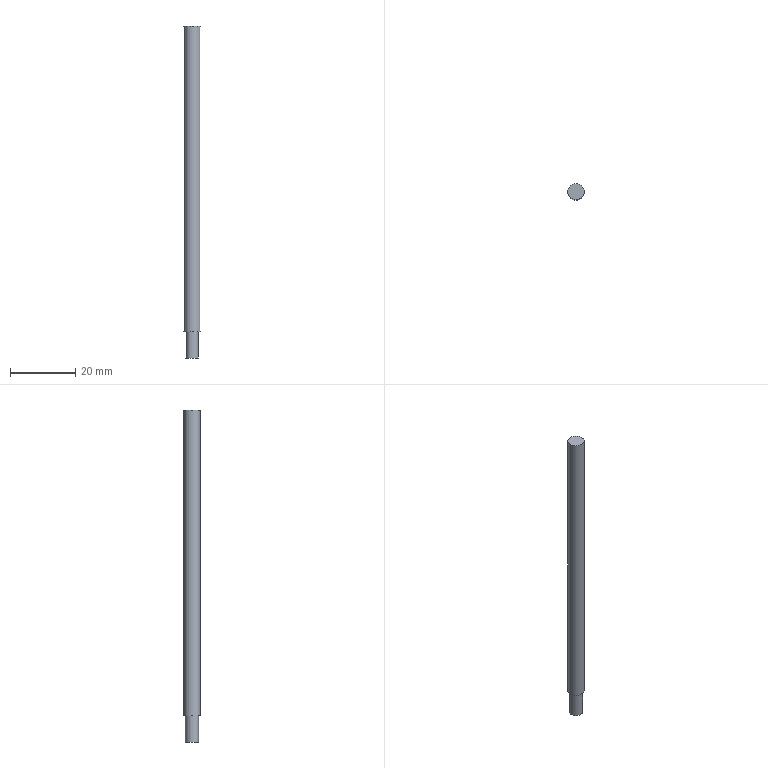Component | NX | PISTON_ROD | 1 solid | 5 faces | box 5 x 5 x 101.5 mm | volume 1936 mm3 | plane 3 | cylinder 2 | commonest cylinder face diameters 5 x1 4 x1
STEP:
#1=CARTESIAN_POINT('',(0.,0.,0.));
#2=DIRECTION('',(0.,0.,1.));
#3=DIRECTION('',(1.,0.,0.));
#4=AXIS2_PLACEMENT_3D('',#1,#2,#3);
#5=CARTESIAN_POINT('',(-0.,-34.5,122.));
#6=VERTEX_POINT('',#5);
#7=CARTESIAN_POINT('',(-0.,-37.,122.));
#8=DIRECTION('',(0.,0.,-1.));
#9=DIRECTION('',(0.,1.,0.));
#10=AXIS2_PLACEMENT_3D('',#7,#8,#9);
#11=CIRCLE('',#10,2.5);
#12=CARTESIAN_POINT('',(-0.,-37.,122.));
#13=DIRECTION('',(0.,0.,1.));
#14=DIRECTION('',(0.,1.,0.));
#15=AXIS2_PLACEMENT_3D('',#12,#13,#14);
#16=PLANE('',#15);
#17=CARTESIAN_POINT('',(2.5,0.));
#18=CARTESIAN_POINT('',(2.5,-4.33));
#19=CARTESIAN_POINT('',(-1.25,-2.165));
#20=CARTESIAN_POINT('',(-5.,-0.));
#21=CARTESIAN_POINT('',(-1.25,2.165));
#22=CARTESIAN_POINT('',(2.5,4.33));
#23=CARTESIAN_POINT('',(2.5,0.));
#24=(BOUNDED_CURVE()B_SPLINE_CURVE(2,(#17,#18,#19,#20,#21,#22,#23),.UNSPECIFIED.,.T.,.F.)B_SPLINE_CURVE_WITH_KNOTS((1,2,2,2,2,1),(-2.094,0.,2.094,4.189,6.283,8.378),.UNSPECIFIED.)CURVE()GEOMETRIC_REPRESENTATION_ITEM()RATIONAL_B_SPLINE_CURVE((1.,0.5,1.,0.5,1.,0.5,1.))REPRESENTATION_ITEM(''));
#25=(GEOMETRIC_REPRESENTATION_CONTEXT(2)PARAMETRIC_REPRESENTATION_CONTEXT()REPRESENTATION_CONTEXT('',''));
#26=DEFINITIONAL_REPRESENTATION('',(#24),#25);
#27=PCURVE('',#16,#26);
#28=CARTESIAN_POINT('',(-0.,-37.,28.5));
#29=DIRECTION('',(0.,0.,1.));
#30=DIRECTION('',(0.,1.,0.));
#31=AXIS2_PLACEMENT_3D('',#28,#29,#30);
#32=CYLINDRICAL_SURFACE('',#31,2.5);
#33=CARTESIAN_POINT('',(6.283,93.5));
#34=DIRECTION('',(-1.,0.));
#35=VECTOR('',#34,1.);
#36=LINE('',#33,#35);
#37=(GEOMETRIC_REPRESENTATION_CONTEXT(2)PARAMETRIC_REPRESENTATION_CONTEXT()REPRESENTATION_CONTEXT('',''));
#38=DEFINITIONAL_REPRESENTATION('',(#36),#37);
#39=PCURVE('',#32,#38);
#40=SURFACE_CURVE('',#11,(#27,#39),.PCURVE_S1.);
#41=EDGE_CURVE('',#6,#6,#40,.T.);
#42=ORIENTED_EDGE('',*,*,#41,.F.);
#43=EDGE_LOOP('',(#42));
#44=FACE_BOUND('',#43,.T.);
#45=ADVANCED_FACE('',(#44),#16,.T.);
#46=CARTESIAN_POINT('',(-0.,-39.,28.5));
#47=VERTEX_POINT('',#46);
#48=CARTESIAN_POINT('',(-0.,-37.,28.5));
#49=DIRECTION('',(0.,0.,-1.));
#50=DIRECTION('',(0.,-1.,0.));
#51=AXIS2_PLACEMENT_3D('',#48,#49,#50);
#52=CIRCLE('',#51,2.);
#53=CARTESIAN_POINT('',(-0.,-37.,28.5));
#54=DIRECTION('',(0.,0.,-1.));
#55=DIRECTION('',(0.,-1.,0.));
#56=AXIS2_PLACEMENT_3D('',#53,#54,#55);
#57=PLANE('',#56);
#58=CARTESIAN_POINT('',(0.,0.));
#59=DIRECTION('',(1.,0.));
#60=AXIS2_PLACEMENT_2D('',#58,#59);
#61=CIRCLE('',#60,2.);
#62=(GEOMETRIC_REPRESENTATION_CONTEXT(2)PARAMETRIC_REPRESENTATION_CONTEXT()REPRESENTATION_CONTEXT('',''));
#63=DEFINITIONAL_REPRESENTATION('',(#61),#62);
#64=PCURVE('',#57,#63);
#65=CARTESIAN_POINT('',(-0.,-37.,28.5));
#66=DIRECTION('',(0.,0.,-1.));
#67=DIRECTION('',(0.,-1.,0.));
#68=AXIS2_PLACEMENT_3D('',#65,#66,#67);
#69=CYLINDRICAL_SURFACE('',#68,2.);
#70=CARTESIAN_POINT('',(0.,0.));
#71=DIRECTION('',(1.,0.));
#72=VECTOR('',#71,1.);
#73=LINE('',#70,#72);
#74=(GEOMETRIC_REPRESENTATION_CONTEXT(2)PARAMETRIC_REPRESENTATION_CONTEXT()REPRESENTATION_CONTEXT('',''));
#75=DEFINITIONAL_REPRESENTATION('',(#73),#74);
#76=PCURVE('',#69,#75);
#77=SURFACE_CURVE('',#52,(#64,#76),.PCURVE_S1.);
#78=EDGE_CURVE('',#47,#47,#77,.T.);
#79=ORIENTED_EDGE('',*,*,#78,.F.);
#80=EDGE_LOOP('',(#79));
#81=FACE_BOUND('',#80,.T.);
#82=CARTESIAN_POINT('',(-0.,-34.5,28.5));
#83=VERTEX_POINT('',#82);
#84=CARTESIAN_POINT('',(-0.,-37.,28.5));
#85=DIRECTION('',(0.,0.,1.));
#86=DIRECTION('',(0.,1.,0.));
#87=AXIS2_PLACEMENT_3D('',#84,#85,#86);
#88=CIRCLE('',#87,2.5);
#89=CARTESIAN_POINT('',(-2.5,0.));
#90=CARTESIAN_POINT('',(-2.5,4.33));
#91=CARTESIAN_POINT('',(1.25,2.165));
#92=CARTESIAN_POINT('',(5.,0.));
#93=CARTESIAN_POINT('',(1.25,-2.165));
#94=CARTESIAN_POINT('',(-2.5,-4.33));
#95=CARTESIAN_POINT('',(-2.5,0.));
#96=(BOUNDED_CURVE()B_SPLINE_CURVE(2,(#89,#90,#91,#92,#93,#94,#95),.UNSPECIFIED.,.T.,.F.)B_SPLINE_CURVE_WITH_KNOTS((1,2,2,2,2,1),(-2.094,0.,2.094,4.189,6.283,8.378),.UNSPECIFIED.)CURVE()GEOMETRIC_REPRESENTATION_ITEM()RATIONAL_B_SPLINE_CURVE((1.,0.5,1.,0.5,1.,0.5,1.))REPRESENTATION_ITEM(''));
#97=(GEOMETRIC_REPRESENTATION_CONTEXT(2)PARAMETRIC_REPRESENTATION_CONTEXT()REPRESENTATION_CONTEXT('',''));
#98=DEFINITIONAL_REPRESENTATION('',(#96),#97);
#99=PCURVE('',#57,#98);
#100=CARTESIAN_POINT('',(0.,0.));
#101=DIRECTION('',(1.,0.));
#102=VECTOR('',#101,1.);
#103=LINE('',#100,#102);
#104=(GEOMETRIC_REPRESENTATION_CONTEXT(2)PARAMETRIC_REPRESENTATION_CONTEXT()REPRESENTATION_CONTEXT('',''));
#105=DEFINITIONAL_REPRESENTATION('',(#103),#104);
#106=PCURVE('',#32,#105);
#107=SURFACE_CURVE('',#88,(#99,#106),.PCURVE_S1.);
#108=EDGE_CURVE('',#83,#83,#107,.T.);
#109=ORIENTED_EDGE('',*,*,#108,.F.);
#110=EDGE_LOOP('',(#109));
#111=FACE_BOUND('',#110,.T.);
#112=ADVANCED_FACE('',(#81,#111),#57,.T.);
#113=ORIENTED_EDGE('',*,*,#41,.T.);
#114=CARTESIAN_POINT('',(-0.,-34.5,28.5));
#115=CARTESIAN_POINT('',(-0.,-34.5,122.));
#116=B_SPLINE_CURVE_WITH_KNOTS('',1,(#114,#115),.UNSPECIFIED.,.F.,.F.,(2,2),(0.,93.5),.PIECEWISE_BEZIER_KNOTS.);
#117=CARTESIAN_POINT('',(0.,0.));
#118=DIRECTION('',(0.,1.));
#119=VECTOR('',#118,1.);
#120=LINE('',#117,#119);
#121=(GEOMETRIC_REPRESENTATION_CONTEXT(2)PARAMETRIC_REPRESENTATION_CONTEXT()REPRESENTATION_CONTEXT('',''));
#122=DEFINITIONAL_REPRESENTATION('',(#120),#121);
#123=PCURVE('',#32,#122);
#124=CARTESIAN_POINT('',(6.283,0.));
#125=DIRECTION('',(0.,1.));
#126=VECTOR('',#125,1.);
#127=LINE('',#124,#126);
#128=(GEOMETRIC_REPRESENTATION_CONTEXT(2)PARAMETRIC_REPRESENTATION_CONTEXT()REPRESENTATION_CONTEXT('',''));
#129=DEFINITIONAL_REPRESENTATION('',(#127),#128);
#130=PCURVE('',#32,#129);
#131=SEAM_CURVE('',#116,(#123,#130),.PCURVE_S1.);
#132=EDGE_CURVE('',#83,#6,#131,.T.);
#133=ORIENTED_EDGE('',*,*,#132,.F.);
#134=ORIENTED_EDGE('',*,*,#108,.T.);
#135=ORIENTED_EDGE('',*,*,#132,.T.);
#136=EDGE_LOOP('',(#113,#133,#134,#135));
#137=FACE_BOUND('',#136,.T.);
#138=ADVANCED_FACE('',(#137),#32,.T.);
#139=CARTESIAN_POINT('',(-0.,-39.,20.5));
#140=VERTEX_POINT('',#139);
#141=CARTESIAN_POINT('',(-0.,-37.,20.5));
#142=DIRECTION('',(0.,0.,-1.));
#143=DIRECTION('',(0.,-1.,0.));
#144=AXIS2_PLACEMENT_3D('',#141,#142,#143);
#145=CIRCLE('',#144,2.);
#146=CARTESIAN_POINT('',(-0.,-37.,20.5));
#147=DIRECTION('',(0.,0.,-1.));
#148=DIRECTION('',(0.,-1.,0.));
#149=AXIS2_PLACEMENT_3D('',#146,#147,#148);
#150=PLANE('',#149);
#151=CARTESIAN_POINT('',(0.,0.));
#152=DIRECTION('',(1.,0.));
#153=AXIS2_PLACEMENT_2D('',#151,#152);
#154=CIRCLE('',#153,2.);
#155=(GEOMETRIC_REPRESENTATION_CONTEXT(2)PARAMETRIC_REPRESENTATION_CONTEXT()REPRESENTATION_CONTEXT('',''));
#156=DEFINITIONAL_REPRESENTATION('',(#154),#155);
#157=PCURVE('',#150,#156);
#158=CARTESIAN_POINT('',(0.,8.));
#159=DIRECTION('',(1.,0.));
#160=VECTOR('',#159,1.);
#161=LINE('',#158,#160);
#162=(GEOMETRIC_REPRESENTATION_CONTEXT(2)PARAMETRIC_REPRESENTATION_CONTEXT()REPRESENTATION_CONTEXT('',''));
#163=DEFINITIONAL_REPRESENTATION('',(#161),#162);
#164=PCURVE('',#69,#163);
#165=SURFACE_CURVE('',#145,(#157,#164),.PCURVE_S1.);
#166=EDGE_CURVE('',#140,#140,#165,.T.);
#167=ORIENTED_EDGE('',*,*,#166,.T.);
#168=EDGE_LOOP('',(#167));
#169=FACE_BOUND('',#168,.T.);
#170=ADVANCED_FACE('',(#169),#150,.T.);
#171=ORIENTED_EDGE('',*,*,#166,.F.);
#172=CARTESIAN_POINT('',(-0.,-39.,28.5));
#173=CARTESIAN_POINT('',(-0.,-39.,20.5));
#174=B_SPLINE_CURVE_WITH_KNOTS('',1,(#172,#173),.UNSPECIFIED.,.F.,.F.,(2,2),(0.,8.),.PIECEWISE_BEZIER_KNOTS.);
#175=CARTESIAN_POINT('',(0.,0.));
#176=DIRECTION('',(0.,1.));
#177=VECTOR('',#176,1.);
#178=LINE('',#175,#177);
#179=(GEOMETRIC_REPRESENTATION_CONTEXT(2)PARAMETRIC_REPRESENTATION_CONTEXT()REPRESENTATION_CONTEXT('',''));
#180=DEFINITIONAL_REPRESENTATION('',(#178),#179);
#181=PCURVE('',#69,#180);
#182=CARTESIAN_POINT('',(6.283,0.));
#183=DIRECTION('',(0.,1.));
#184=VECTOR('',#183,1.);
#185=LINE('',#182,#184);
#186=(GEOMETRIC_REPRESENTATION_CONTEXT(2)PARAMETRIC_REPRESENTATION_CONTEXT()REPRESENTATION_CONTEXT('',''));
#187=DEFINITIONAL_REPRESENTATION('',(#185),#186);
#188=PCURVE('',#69,#187);
#189=SEAM_CURVE('',#174,(#181,#188),.PCURVE_S1.);
#190=EDGE_CURVE('',#47,#140,#189,.T.);
#191=ORIENTED_EDGE('',*,*,#190,.F.);
#192=ORIENTED_EDGE('',*,*,#78,.T.);
#193=ORIENTED_EDGE('',*,*,#190,.T.);
#194=EDGE_LOOP('',(#171,#191,#192,#193));
#195=FACE_BOUND('',#194,.T.);
#196=ADVANCED_FACE('',(#195),#69,.T.);
#197=CLOSED_SHELL('',(#45,#112,#138,#170,#196));
#198=MANIFOLD_SOLID_BREP('',#197);
#199=(LENGTH_UNIT()NAMED_UNIT(*)SI_UNIT(.MILLI.,.METRE.));
#200=UNCERTAINTY_MEASURE_WITH_UNIT(LENGTH_MEASURE(0.00001),#199,'','');
#201=(NAMED_UNIT(*)PLANE_ANGLE_UNIT()SI_UNIT($,.RADIAN.));
#202=(NAMED_UNIT(*)SI_UNIT($,.STERADIAN.)SOLID_ANGLE_UNIT());
#203=(GEOMETRIC_REPRESENTATION_CONTEXT(3)GLOBAL_UNCERTAINTY_ASSIGNED_CONTEXT((#200))GLOBAL_UNIT_ASSIGNED_CONTEXT((#199,#201,#202))REPRESENTATION_CONTEXT('',''));
#204=ADVANCED_BREP_SHAPE_REPRESENTATION('',(#4,#198),#203);